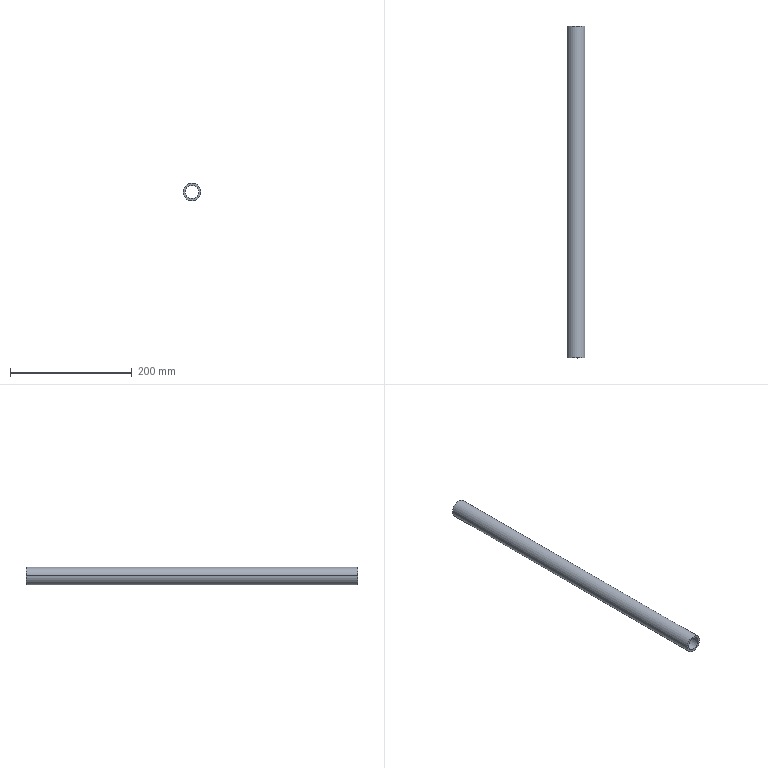Component | SolidWorks | YC1-250-04BalancerAssembly#16673-1_YC1-250-04-13#16673Sleeve-1 | 1 solid | 6 faces | box 29 x 545 x 29 mm | volume 152811 mm3 | cylinder 4 | plane 2 | commonest cylinder face diameters 29 x2 22 x2 | material Plain Carbon Steel
STEP:
#1=COLOUR_RGB('',0.7922,0.8196,0.9333);
#2=FILL_AREA_STYLE_COLOUR('',#1);
#3=FILL_AREA_STYLE('',(#2));
#4=SURFACE_STYLE_FILL_AREA(#3);
#5=SURFACE_SIDE_STYLE('',(#4));
#6=SURFACE_STYLE_USAGE(.BOTH.,#5);
#7=PRESENTATION_STYLE_ASSIGNMENT((#6));
#8=CARTESIAN_POINT('',(-22.272,178.937,4.731));
#9=VERTEX_POINT('',#8);
#10=CARTESIAN_POINT('',(-23.414,178.937,4.734));
#11=VERTEX_POINT('',#10);
#12=CARTESIAN_POINT('',(-22.843,178.937,4.733));
#13=DIRECTION('',(-0.,-1.,0.));
#14=DIRECTION('',(1.,0.,-0.00245));
#15=AXIS2_PLACEMENT_3D('',#12,#13,#14);
#16=CIRCLE('',#15,0.5709);
#17=EDGE_CURVE('',#9,#11,#16,.T.);
#18=ORIENTED_EDGE('',*,*,#17,.T.);
#19=CARTESIAN_POINT('',(-23.414,157.48,4.734));
#20=VERTEX_POINT('',#19);
#21=CARTESIAN_POINT('',(-23.414,178.937,4.734));
#22=DIRECTION('',(-0.,-1.,0.));
#23=VECTOR('',#22,39.37);
#24=LINE('',#21,#23);
#25=EDGE_CURVE('',#11,#20,#24,.T.);
#26=ORIENTED_EDGE('',*,*,#25,.T.);
#27=CARTESIAN_POINT('',(-22.272,157.48,4.731));
#28=VERTEX_POINT('',#27);
#29=CARTESIAN_POINT('',(-22.843,157.48,4.733));
#30=DIRECTION('',(0.,1.,-0.));
#31=DIRECTION('',(1.,0.,-0.00245));
#32=AXIS2_PLACEMENT_3D('',#29,#30,#31);
#33=CIRCLE('',#32,0.5709);
#34=EDGE_CURVE('',#20,#28,#33,.T.);
#35=ORIENTED_EDGE('',*,*,#34,.T.);
#36=CARTESIAN_POINT('',(-22.272,178.937,4.731));
#37=DIRECTION('',(-0.,-1.,0.));
#38=VECTOR('',#37,39.37);
#39=LINE('',#36,#38);
#40=EDGE_CURVE('',#9,#28,#39,.T.);
#41=ORIENTED_EDGE('',*,*,#40,.F.);
#42=EDGE_LOOP('',(#18,#26,#35,#41));
#43=FACE_OUTER_BOUND('',#42,.T.);
#44=CARTESIAN_POINT('',(-22.843,178.937,4.733));
#45=DIRECTION('',(-0.,-1.,0.));
#46=DIRECTION('',(1.,0.,-0.00245));
#47=AXIS2_PLACEMENT_3D('',#44,#45,#46);
#48=CYLINDRICAL_SURFACE('',#47,0.5709);
#49=ADVANCED_FACE('',(#43),#48,.T.);
#50=CARTESIAN_POINT('',(-23.276,178.937,4.734));
#51=VERTEX_POINT('',#50);
#52=CARTESIAN_POINT('',(-22.41,178.937,4.732));
#53=VERTEX_POINT('',#52);
#54=CARTESIAN_POINT('',(-22.843,178.937,4.733));
#55=DIRECTION('',(-0.,-1.,0.));
#56=DIRECTION('',(1.,0.,-0.00245));
#57=AXIS2_PLACEMENT_3D('',#54,#55,#56);
#58=CIRCLE('',#57,0.4331);
#59=EDGE_CURVE('',#51,#53,#58,.T.);
#60=ORIENTED_EDGE('',*,*,#59,.F.);
#61=CARTESIAN_POINT('',(-23.276,157.48,4.734));
#62=VERTEX_POINT('',#61);
#63=CARTESIAN_POINT('',(-23.276,178.937,4.734));
#64=DIRECTION('',(-0.,-1.,0.));
#65=VECTOR('',#64,39.37);
#66=LINE('',#63,#65);
#67=EDGE_CURVE('',#51,#62,#66,.T.);
#68=ORIENTED_EDGE('',*,*,#67,.T.);
#69=CARTESIAN_POINT('',(-22.41,157.48,4.732));
#70=VERTEX_POINT('',#69);
#71=CARTESIAN_POINT('',(-22.843,157.48,4.733));
#72=DIRECTION('',(-0.,-1.,0.));
#73=DIRECTION('',(1.,0.,-0.00245));
#74=AXIS2_PLACEMENT_3D('',#71,#72,#73);
#75=CIRCLE('',#74,0.4331);
#76=EDGE_CURVE('',#62,#70,#75,.T.);
#77=ORIENTED_EDGE('',*,*,#76,.T.);
#78=CARTESIAN_POINT('',(-22.41,178.937,4.732));
#79=DIRECTION('',(-0.,-1.,0.));
#80=VECTOR('',#79,39.37);
#81=LINE('',#78,#80);
#82=EDGE_CURVE('',#53,#70,#81,.T.);
#83=ORIENTED_EDGE('',*,*,#82,.F.);
#84=EDGE_LOOP('',(#60,#68,#77,#83));
#85=FACE_OUTER_BOUND('',#84,.T.);
#86=CARTESIAN_POINT('',(-22.843,178.937,4.733));
#87=DIRECTION('',(-0.,-1.,0.));
#88=DIRECTION('',(1.,0.,-0.00245));
#89=AXIS2_PLACEMENT_3D('',#86,#87,#88);
#90=CYLINDRICAL_SURFACE('',#89,0.4331);
#91=ADVANCED_FACE('',(#85),#90,.F.);
#92=ORIENTED_EDGE('',*,*,#25,.F.);
#93=CARTESIAN_POINT('',(-22.843,178.937,4.733));
#94=DIRECTION('',(-0.,-1.,0.));
#95=DIRECTION('',(1.,0.,-0.00245));
#96=AXIS2_PLACEMENT_3D('',#93,#94,#95);
#97=CIRCLE('',#96,0.5709);
#98=EDGE_CURVE('',#11,#9,#97,.T.);
#99=ORIENTED_EDGE('',*,*,#98,.T.);
#100=ORIENTED_EDGE('',*,*,#40,.T.);
#101=CARTESIAN_POINT('',(-22.843,157.48,4.733));
#102=DIRECTION('',(0.,1.,-0.));
#103=DIRECTION('',(1.,0.,-0.00245));
#104=AXIS2_PLACEMENT_3D('',#101,#102,#103);
#105=CIRCLE('',#104,0.5709);
#106=EDGE_CURVE('',#28,#20,#105,.T.);
#107=ORIENTED_EDGE('',*,*,#106,.T.);
#108=EDGE_LOOP('',(#92,#99,#100,#107));
#109=FACE_OUTER_BOUND('',#108,.T.);
#110=CARTESIAN_POINT('',(-22.843,178.937,4.733));
#111=DIRECTION('',(-0.,-1.,0.));
#112=DIRECTION('',(1.,0.,-0.00245));
#113=AXIS2_PLACEMENT_3D('',#110,#111,#112);
#114=CYLINDRICAL_SURFACE('',#113,0.5709);
#115=ADVANCED_FACE('',(#109),#114,.T.);
#116=CARTESIAN_POINT('',(-22.843,157.48,4.733));
#117=DIRECTION('',(-0.,-1.,0.));
#118=DIRECTION('',(1.,0.,-0.00245));
#119=AXIS2_PLACEMENT_3D('',#116,#117,#118);
#120=CIRCLE('',#119,0.4331);
#121=EDGE_CURVE('',#70,#62,#120,.T.);
#122=ORIENTED_EDGE('',*,*,#121,.F.);
#123=ORIENTED_EDGE('',*,*,#76,.F.);
#124=EDGE_LOOP('',(#122,#123));
#125=FACE_BOUND('',#124,.T.);
#126=ORIENTED_EDGE('',*,*,#106,.F.);
#127=ORIENTED_EDGE('',*,*,#34,.F.);
#128=EDGE_LOOP('',(#126,#127));
#129=FACE_OUTER_BOUND('',#128,.T.);
#130=CARTESIAN_POINT('',(-22.843,157.48,4.733));
#131=DIRECTION('',(0.,1.,-0.));
#132=DIRECTION('',(-1.,0.,0.00245));
#133=AXIS2_PLACEMENT_3D('',#130,#131,#132);
#134=PLANE('',#133);
#135=ADVANCED_FACE('',(#125,#129),#134,.F.);
#136=CARTESIAN_POINT('',(-22.843,178.937,4.733));
#137=DIRECTION('',(-0.,-1.,0.));
#138=DIRECTION('',(1.,0.,-0.00245));
#139=AXIS2_PLACEMENT_3D('',#136,#137,#138);
#140=CIRCLE('',#139,0.4331);
#141=EDGE_CURVE('',#53,#51,#140,.T.);
#142=ORIENTED_EDGE('',*,*,#141,.T.);
#143=ORIENTED_EDGE('',*,*,#59,.T.);
#144=EDGE_LOOP('',(#142,#143));
#145=FACE_BOUND('',#144,.T.);
#146=ORIENTED_EDGE('',*,*,#17,.F.);
#147=ORIENTED_EDGE('',*,*,#98,.F.);
#148=EDGE_LOOP('',(#146,#147));
#149=FACE_OUTER_BOUND('',#148,.T.);
#150=CARTESIAN_POINT('',(-22.843,178.937,4.733));
#151=DIRECTION('',(0.,1.,-0.));
#152=DIRECTION('',(-1.,0.,0.00245));
#153=AXIS2_PLACEMENT_3D('',#150,#151,#152);
#154=PLANE('',#153);
#155=ADVANCED_FACE('',(#145,#149),#154,.T.);
#156=ORIENTED_EDGE('',*,*,#67,.F.);
#157=ORIENTED_EDGE('',*,*,#141,.F.);
#158=ORIENTED_EDGE('',*,*,#82,.T.);
#159=ORIENTED_EDGE('',*,*,#121,.T.);
#160=EDGE_LOOP('',(#156,#157,#158,#159));
#161=FACE_OUTER_BOUND('',#160,.T.);
#162=CARTESIAN_POINT('',(-22.843,178.937,4.733));
#163=DIRECTION('',(-0.,-1.,0.));
#164=DIRECTION('',(1.,0.,-0.00245));
#165=AXIS2_PLACEMENT_3D('',#162,#163,#164);
#166=CYLINDRICAL_SURFACE('',#165,0.4331);
#167=ADVANCED_FACE('',(#161),#166,.F.);
#168=CLOSED_SHELL('',(#49,#91,#115,#135,#155,#167));
#169=MANIFOLD_SOLID_BREP('',#168);
#170=STYLED_ITEM('',(#7),#169);
#171=PRESENTATION_LAYER_ASSIGNMENT('','',(#170));
#172=CARTESIAN_POINT('',(0.,0.,0.));
#173=DIRECTION('',(0.,0.,1.));
#174=DIRECTION('',(1.,0.,0.));
#175=AXIS2_PLACEMENT_3D('',#172,#173,#174);
#176=(LENGTH_UNIT()NAMED_UNIT(*)SI_UNIT($,.METRE.));
#177=LENGTH_MEASURE_WITH_UNIT(LENGTH_MEASURE(0.0254),#176);
#178=DIMENSIONAL_EXPONENTS(1.,0.,0.,0.,0.,0.,0.);
#179=(CONVERSION_BASED_UNIT('',#177)LENGTH_UNIT()NAMED_UNIT(#178));
#180=UNCERTAINTY_MEASURE_WITH_UNIT(LENGTH_MEASURE(0.00001),#179,'','');
#181=(NAMED_UNIT(*)PLANE_ANGLE_UNIT()SI_UNIT($,.RADIAN.));
#182=(NAMED_UNIT(*)SI_UNIT($,.STERADIAN.)SOLID_ANGLE_UNIT());
#183=(GEOMETRIC_REPRESENTATION_CONTEXT(3)GLOBAL_UNCERTAINTY_ASSIGNED_CONTEXT((#180))GLOBAL_UNIT_ASSIGNED_CONTEXT((#179,#181,#182))REPRESENTATION_CONTEXT('',''));
#184=ADVANCED_BREP_SHAPE_REPRESENTATION('',(#169,#175),#183);
#185=(LENGTH_UNIT()NAMED_UNIT(*)SI_UNIT($,.METRE.));
#186=LENGTH_MEASURE_WITH_UNIT(LENGTH_MEASURE(0.0254),#185);
#187=DIMENSIONAL_EXPONENTS(1.,0.,0.,0.,0.,0.,0.);
#188=(CONVERSION_BASED_UNIT('',#186)LENGTH_UNIT()NAMED_UNIT(#187));
#189=UNCERTAINTY_MEASURE_WITH_UNIT(LENGTH_MEASURE(0.00001),#188,'','');
#190=(NAMED_UNIT(*)PLANE_ANGLE_UNIT()SI_UNIT($,.RADIAN.));
#191=(NAMED_UNIT(*)SI_UNIT($,.STERADIAN.)SOLID_ANGLE_UNIT());
#192=(GEOMETRIC_REPRESENTATION_CONTEXT(3)GLOBAL_UNCERTAINTY_ASSIGNED_CONTEXT((#189))GLOBAL_UNIT_ASSIGNED_CONTEXT((#188,#190,#191))REPRESENTATION_CONTEXT('',''));
#193=MECHANICAL_DESIGN_GEOMETRIC_PRESENTATION_REPRESENTATION('',(#170),#192);